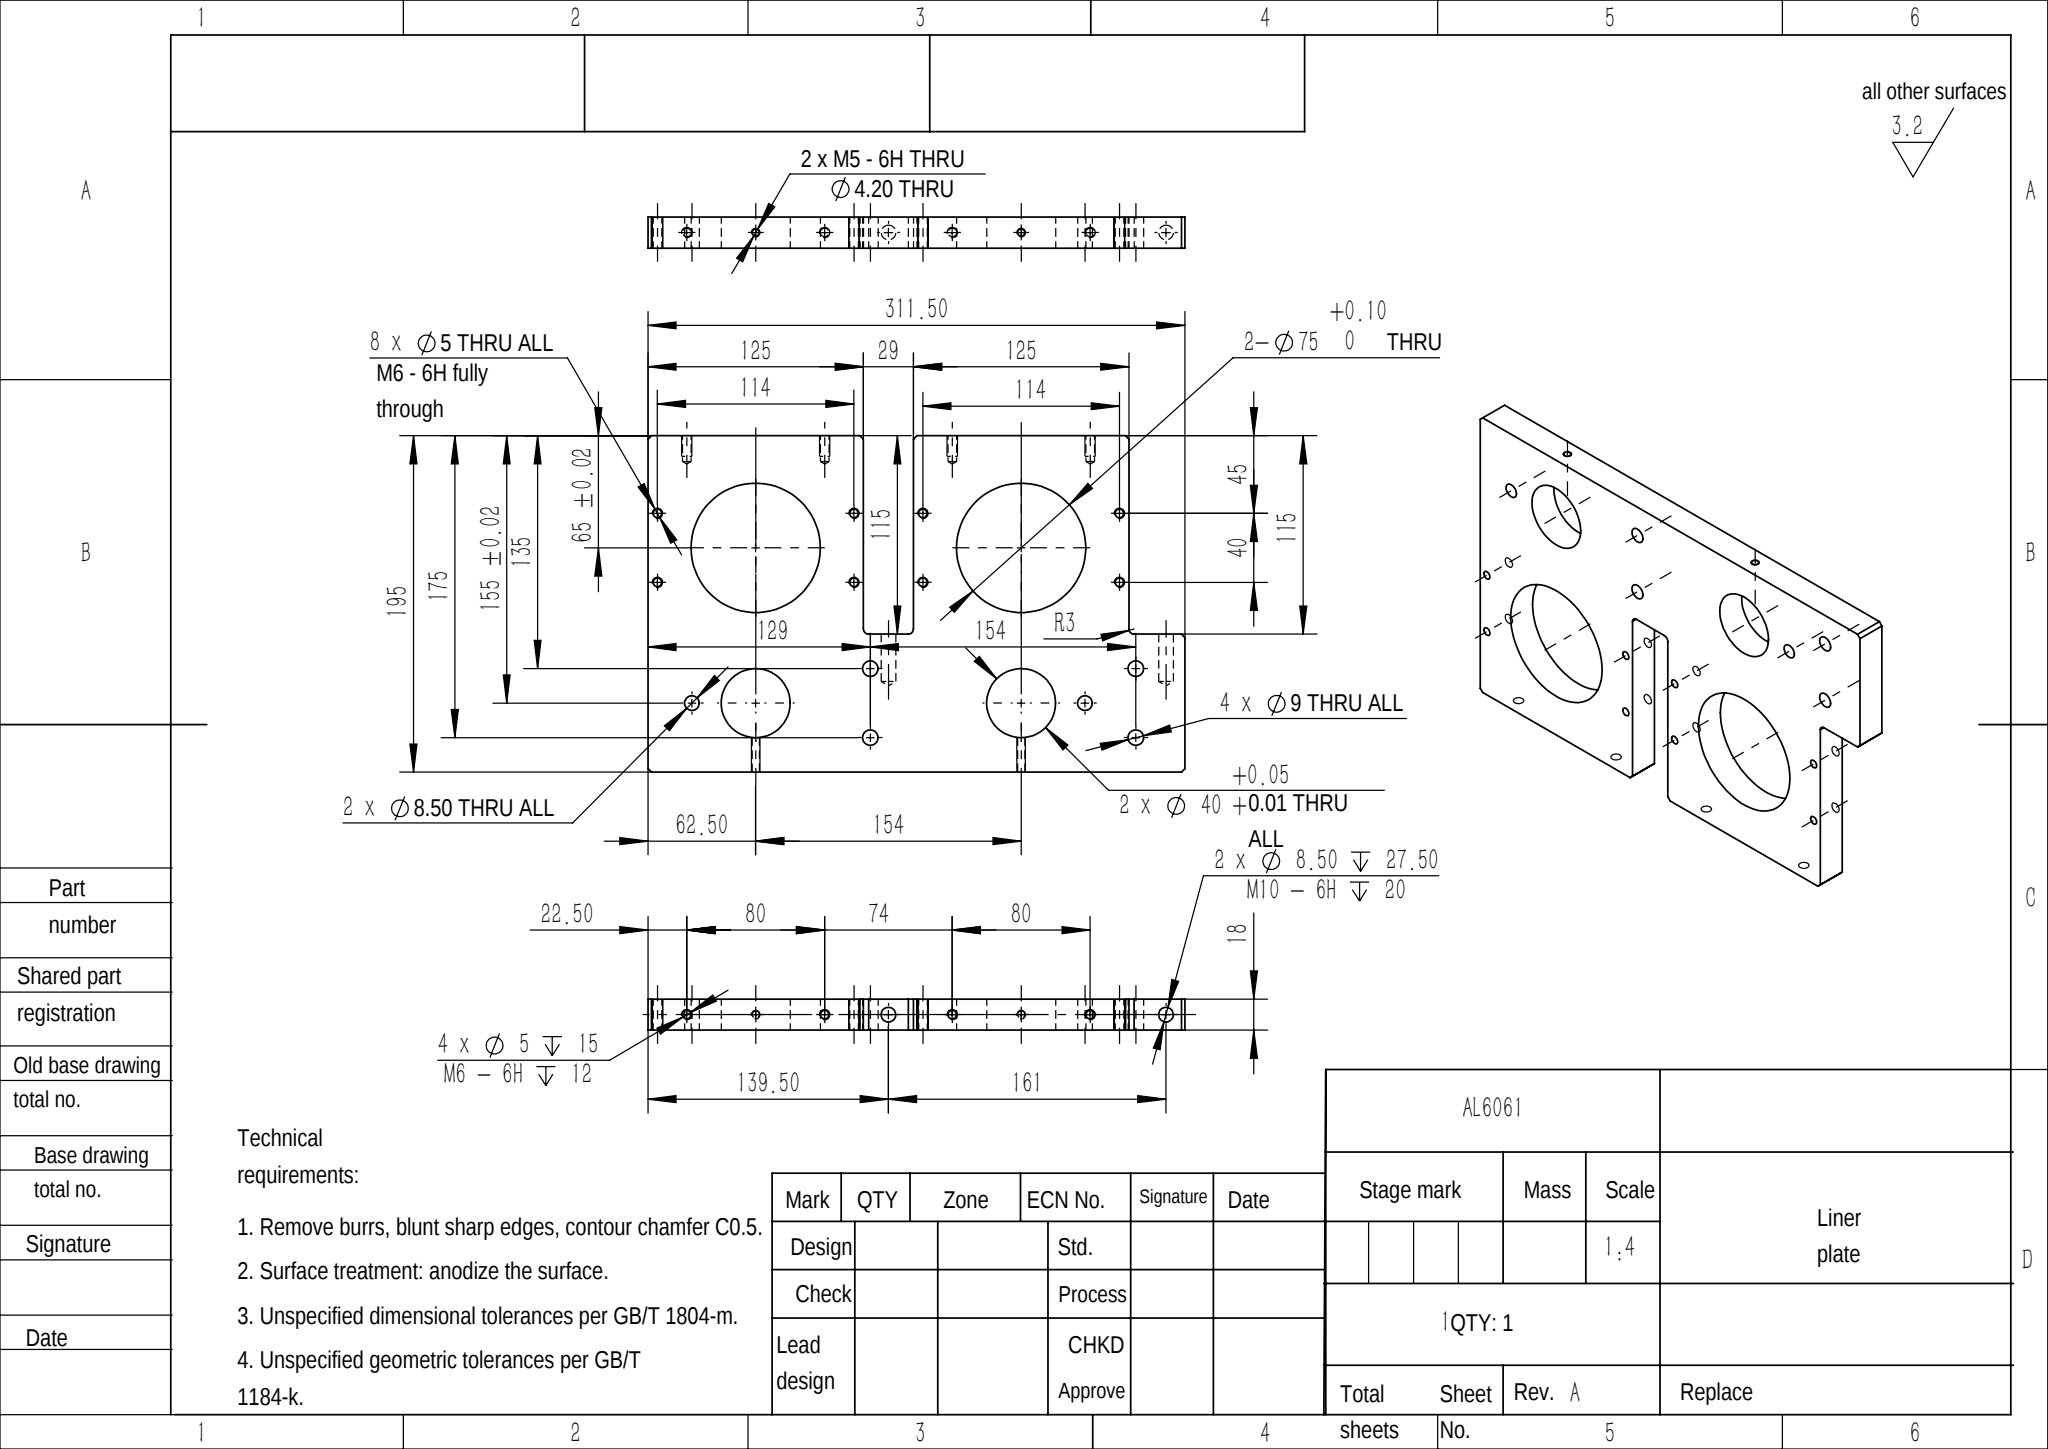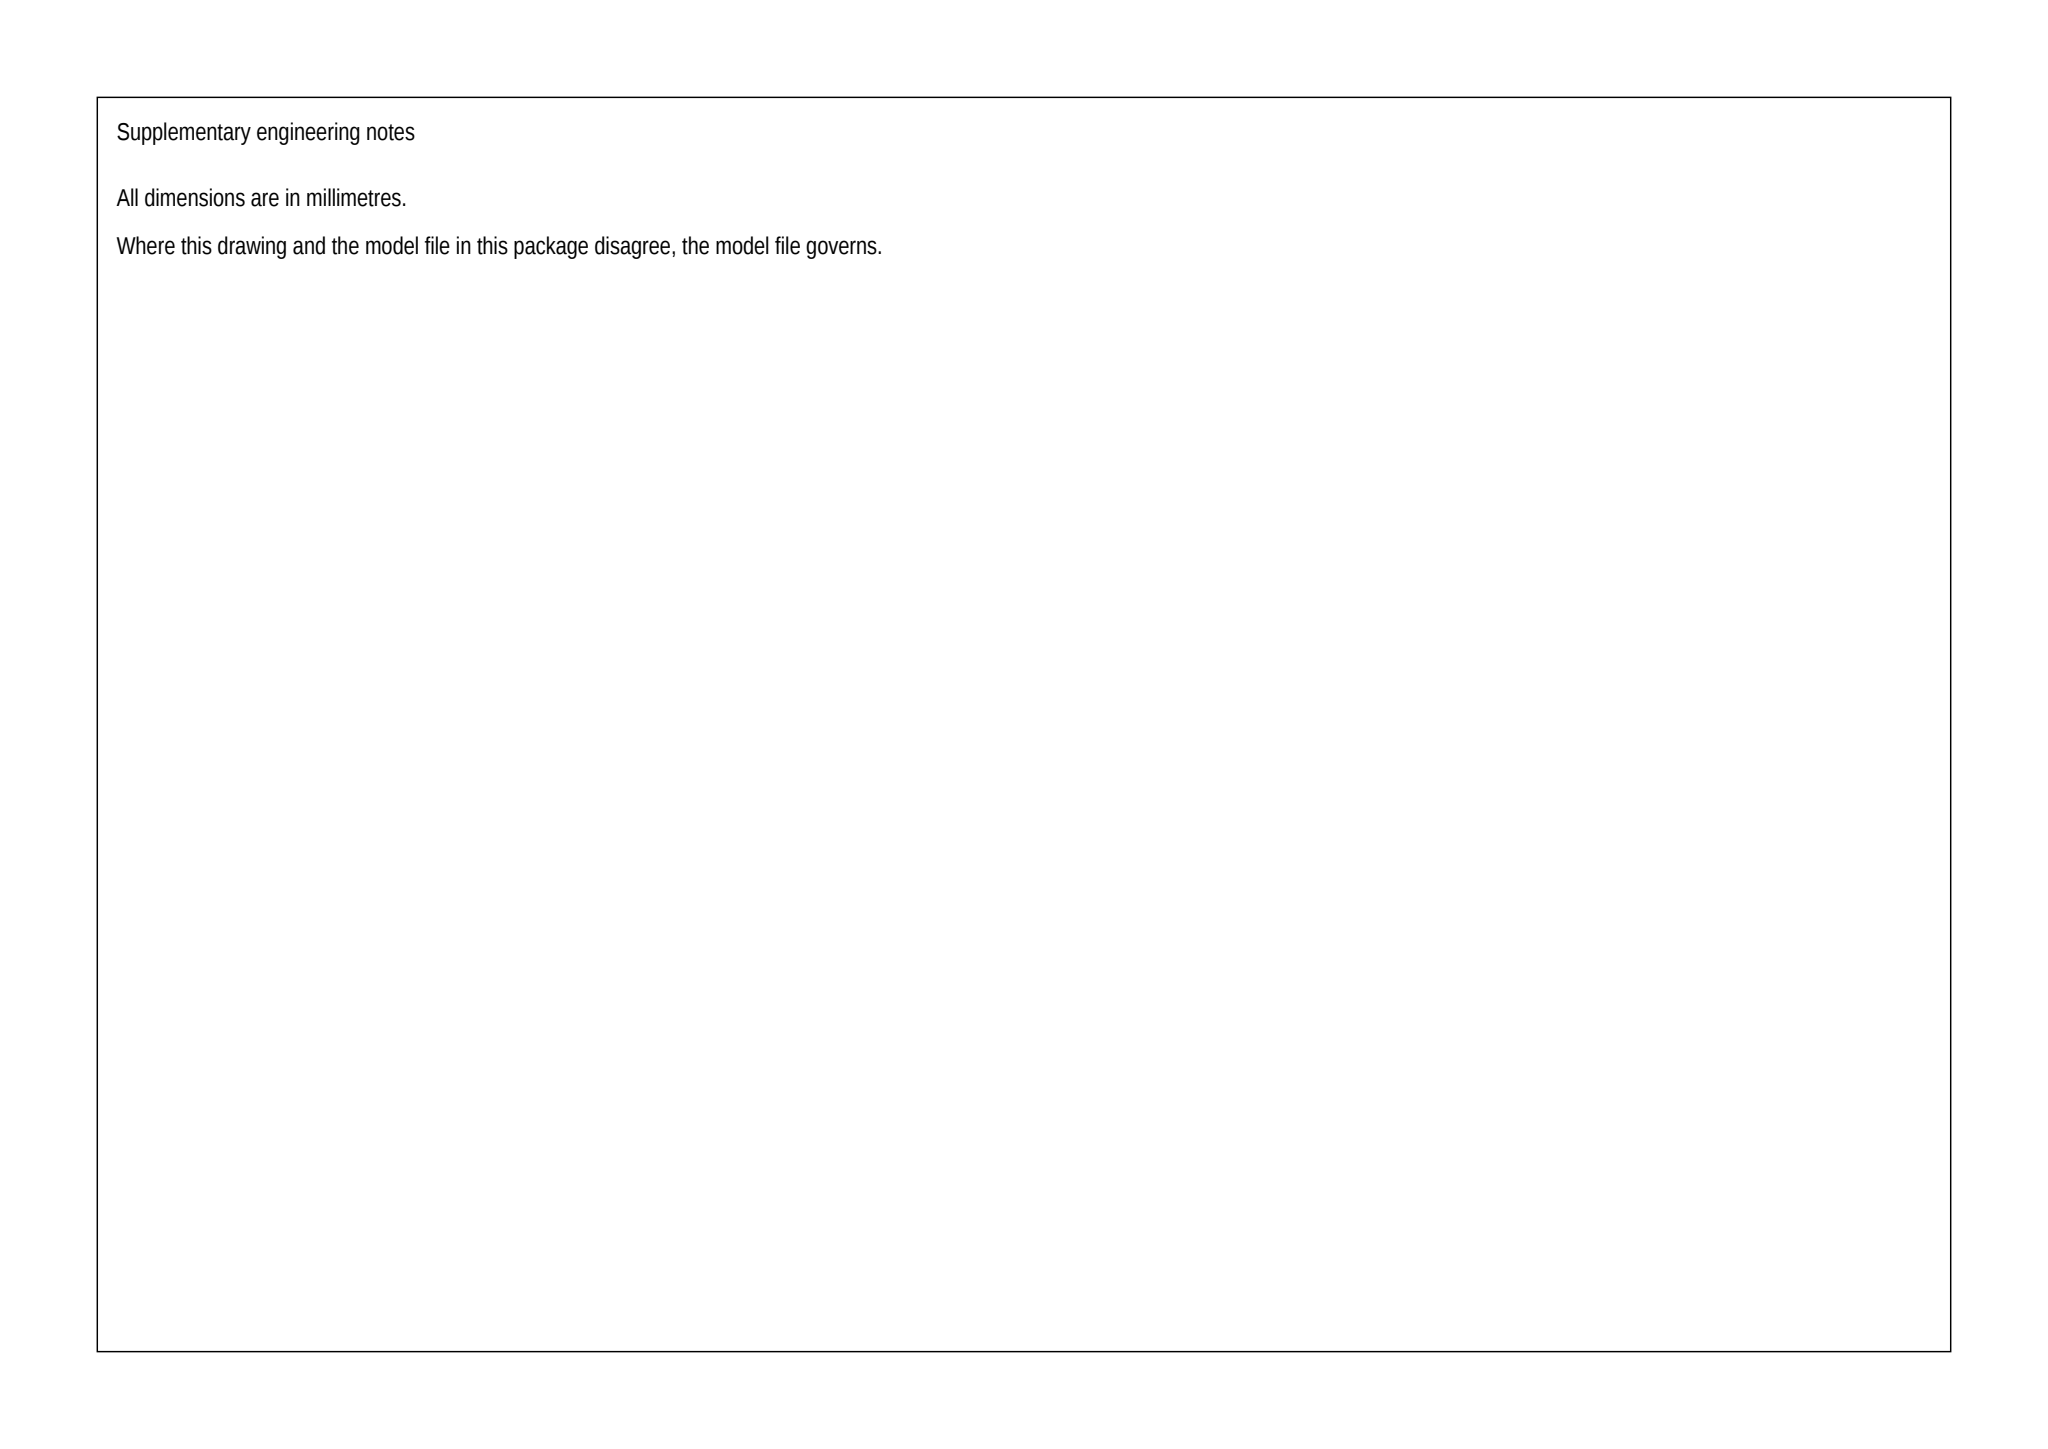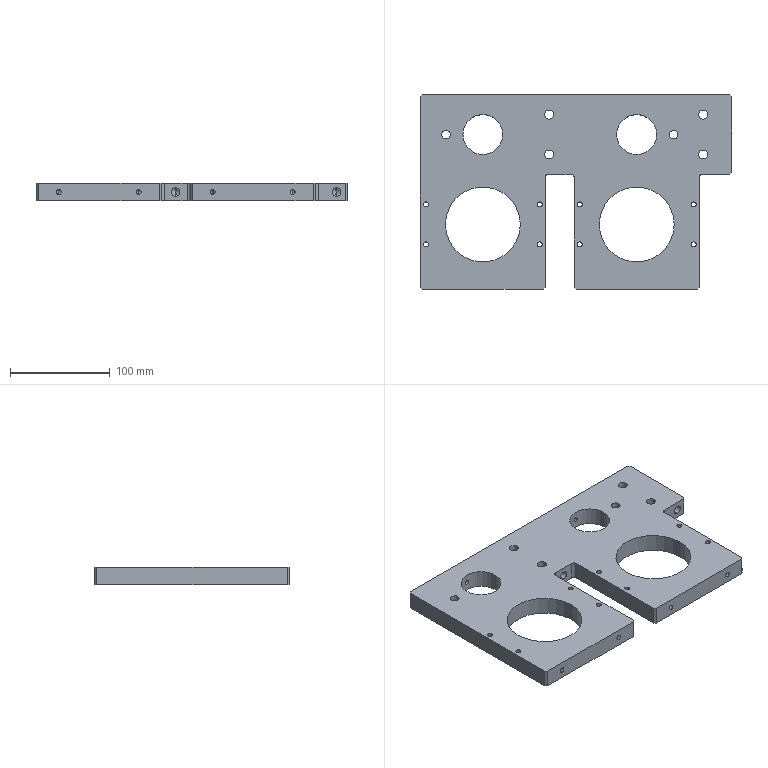Part | SolidWorks | mm | material AL6061 | 1 solid | 86 faces | box 311.5 x 195 x 18 mm | volume 747189 mm3 | cylinder 55 | plane 19 | cone 12 | commonest cylinder face diameters 5 x24 8.5 x8 9 x8 4.2 x4 75 x4 40 x4 6 x3